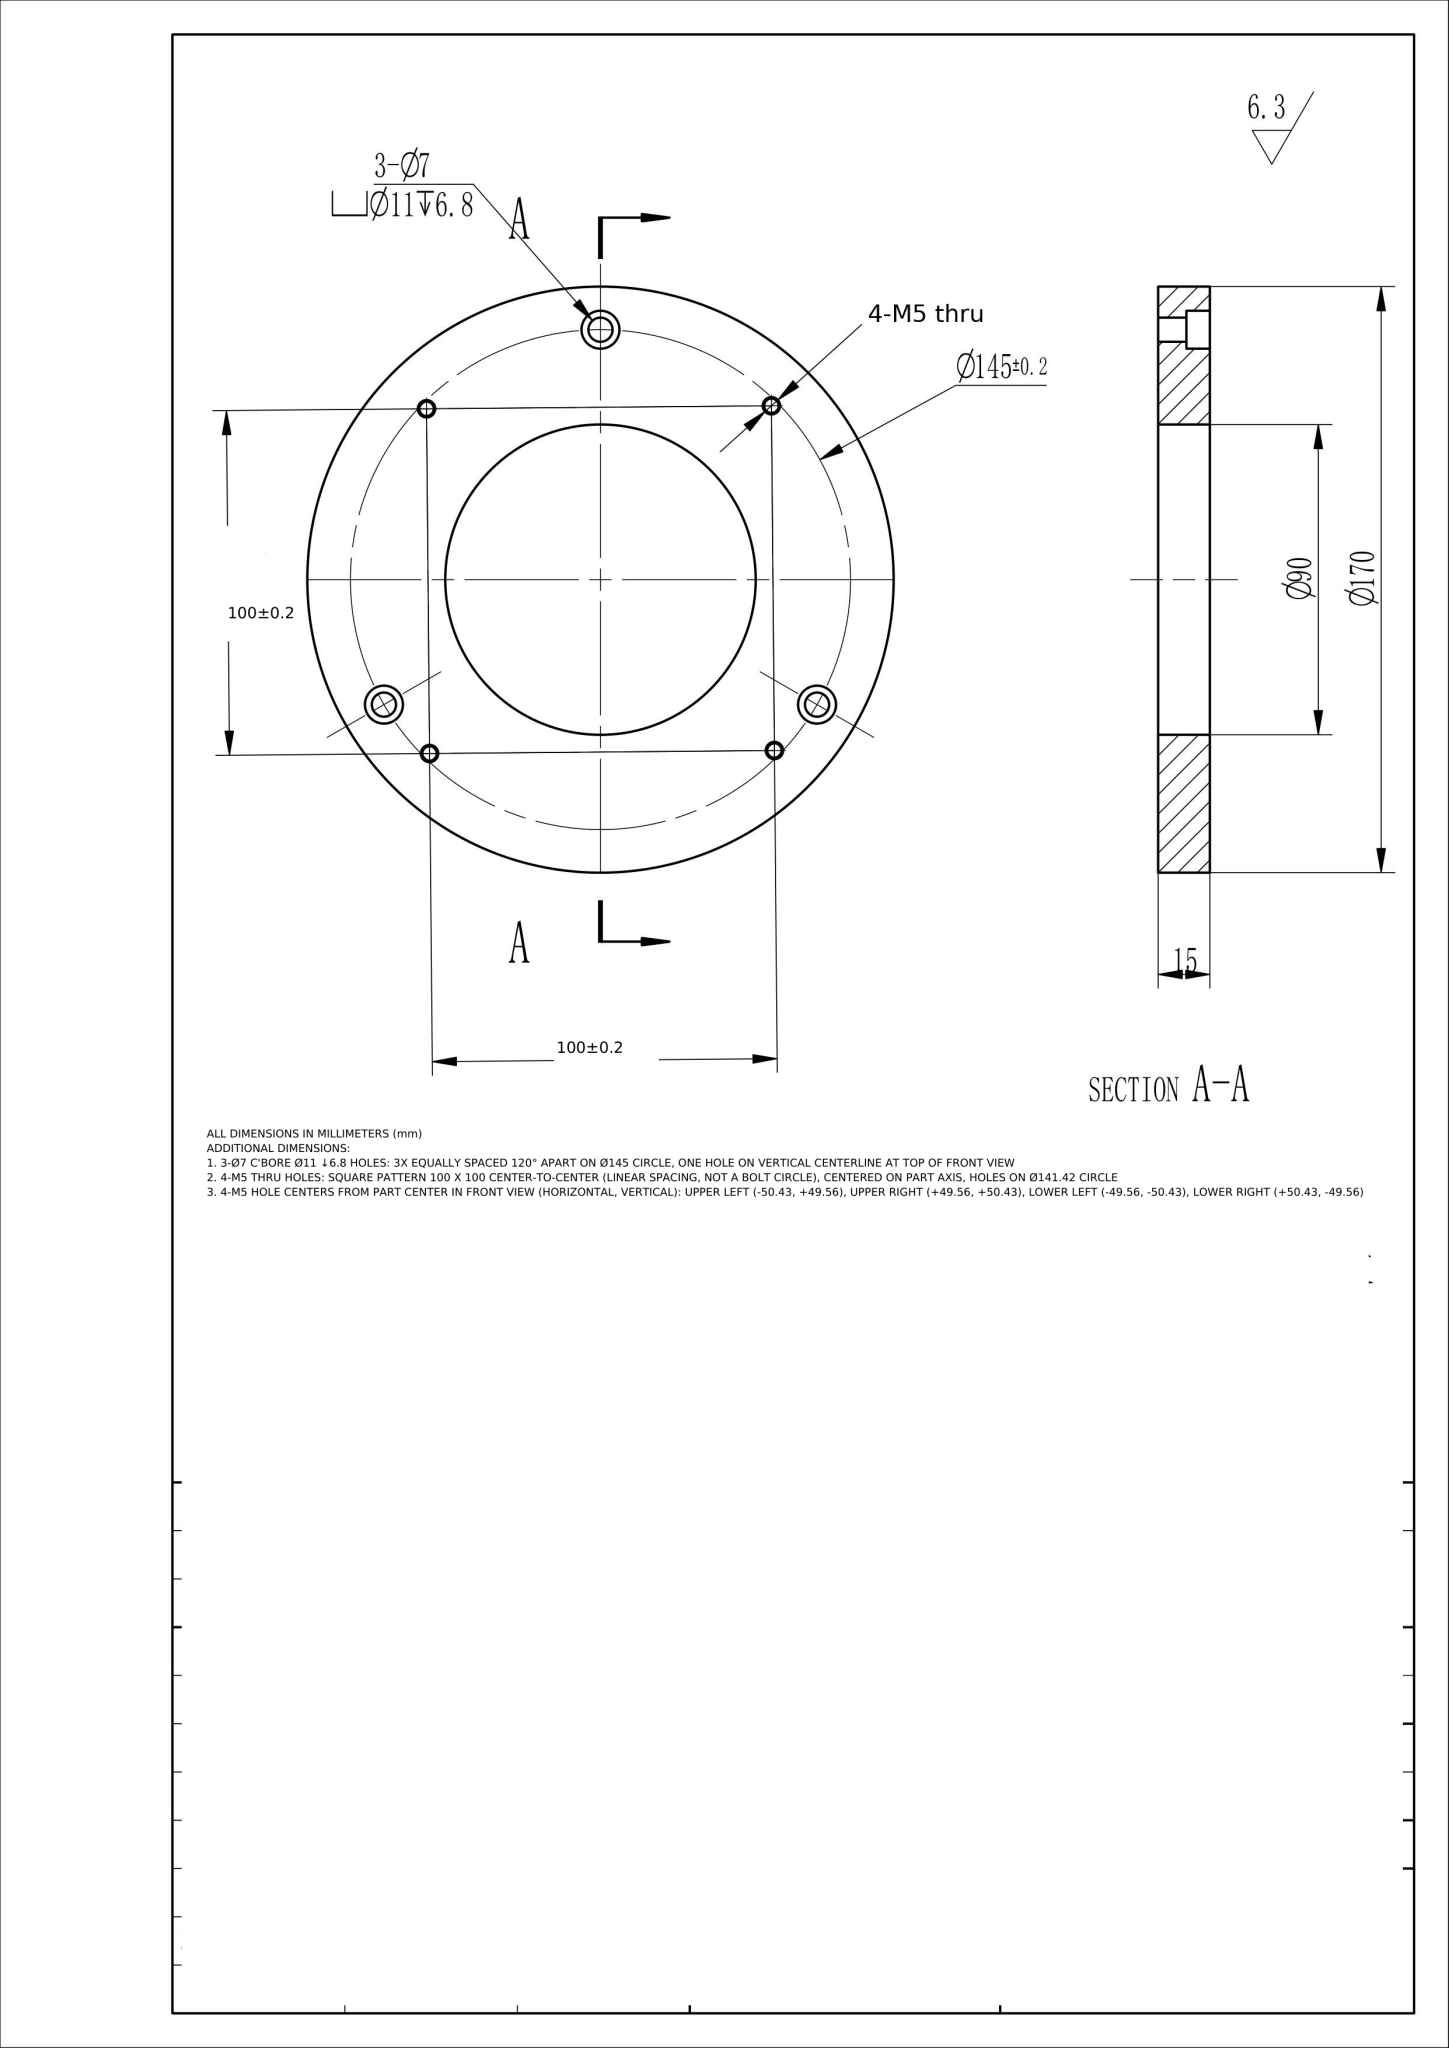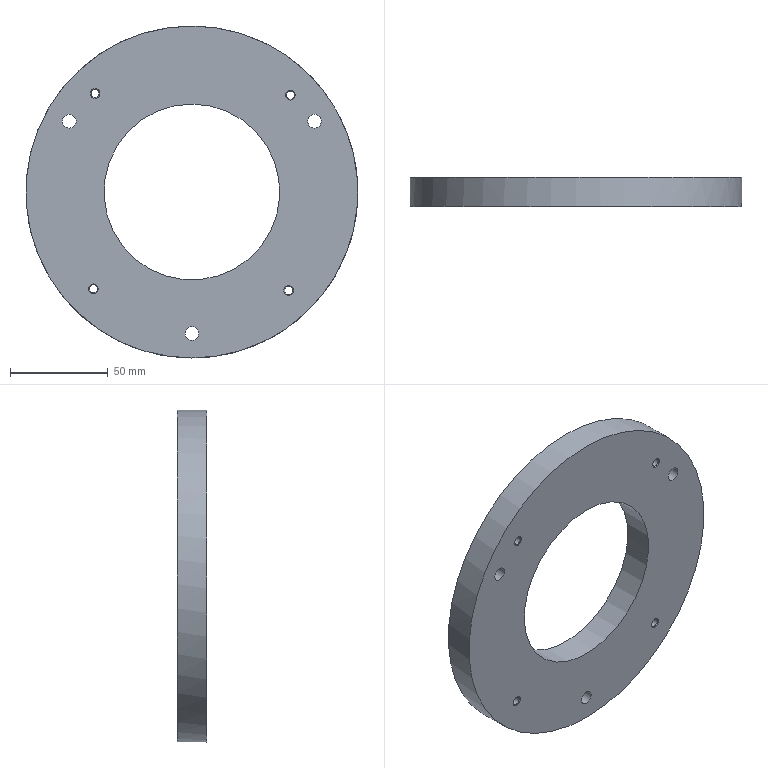Part | NX | mm | 1 solid | 25 faces | box 170 x 15 x 170 mm | volume 241319 mm3 | cylinder 12 | cone 8 | plane 5 | commonest cylinder face diameters 4.2 x4 7 x3 11 x3 170 x1 90 x1
STEP:
#1=CARTESIAN_POINT('',(0.,0.,0.));
#2=DIRECTION('',(0.,0.,1.));
#3=DIRECTION('',(1.,0.,0.));
#4=AXIS2_PLACEMENT_3D('',#1,#2,#3);
#5=(LENGTH_UNIT()NAMED_UNIT(*)SI_UNIT(.MILLI.,.METRE.));
#6=UNCERTAINTY_MEASURE_WITH_UNIT(LENGTH_MEASURE(0.00002),#5,'','');
#7=(NAMED_UNIT(*)PLANE_ANGLE_UNIT()SI_UNIT($,.RADIAN.));
#8=PLANE_ANGLE_MEASURE_WITH_UNIT(PLANE_ANGLE_MEASURE(0.01745),#7);
#9=DIMENSIONAL_EXPONENTS(0.,0.,0.,0.,0.,0.,0.);
#10=(CONVERSION_BASED_UNIT('',#8)NAMED_UNIT(#9)PLANE_ANGLE_UNIT());
#11=(NAMED_UNIT(*)SI_UNIT($,.STERADIAN.)SOLID_ANGLE_UNIT());
#12=(GEOMETRIC_REPRESENTATION_CONTEXT(3)GLOBAL_UNCERTAINTY_ASSIGNED_CONTEXT((#6))GLOBAL_UNIT_ASSIGNED_CONTEXT((#5,#10,#11))REPRESENTATION_CONTEXT('',''));
#13=SHAPE_REPRESENTATION('',(#4),#12);
#14=CARTESIAN_POINT('',(0.,409.,85.));
#15=VERTEX_POINT('',#14);
#16=CARTESIAN_POINT('',(0.,409.,0.));
#17=DIRECTION('',(0.,1.,0.));
#18=DIRECTION('',(0.,0.,1.));
#19=AXIS2_PLACEMENT_3D('',#16,#17,#18);
#20=CIRCLE('',#19,85.);
#21=EDGE_CURVE('',#15,#15,#20,.T.);
#22=ORIENTED_EDGE('',*,*,#21,.T.);
#23=EDGE_LOOP('',(#22));
#24=FACE_BOUND('',#23,.T.);
#25=CARTESIAN_POINT('',(85.,424.,0.));
#26=VERTEX_POINT('',#25);
#27=CARTESIAN_POINT('',(0.,424.,0.));
#28=DIRECTION('',(0.,1.,0.));
#29=DIRECTION('',(1.,0.,0.));
#30=AXIS2_PLACEMENT_3D('',#27,#28,#29);
#31=CIRCLE('',#30,85.);
#32=EDGE_CURVE('',#26,#26,#31,.T.);
#33=ORIENTED_EDGE('',*,*,#32,.F.);
#34=EDGE_LOOP('',(#33));
#35=FACE_BOUND('',#34,.T.);
#36=CARTESIAN_POINT('',(0.,414.,0.));
#37=DIRECTION('',(0.,1.,0.));
#38=DIRECTION('',(0.,0.,1.));
#39=AXIS2_PLACEMENT_3D('',#36,#37,#38);
#40=CYLINDRICAL_SURFACE('',#39,85.);
#41=ADVANCED_FACE('',(#24,#35),#40,.T.);
#42=CARTESIAN_POINT('',(50.434,409.,52.062));
#43=VERTEX_POINT('',#42);
#44=CARTESIAN_POINT('',(50.434,409.,49.562));
#45=DIRECTION('',(0.,1.,0.));
#46=DIRECTION('',(0.,0.,1.));
#47=AXIS2_PLACEMENT_3D('',#44,#45,#46);
#48=CIRCLE('',#47,2.5);
#49=EDGE_CURVE('',#43,#43,#48,.T.);
#50=ORIENTED_EDGE('',*,*,#49,.T.);
#51=EDGE_LOOP('',(#50));
#52=FACE_BOUND('',#51,.T.);
#53=CARTESIAN_POINT('',(49.562,409.,-47.934));
#54=VERTEX_POINT('',#53);
#55=CARTESIAN_POINT('',(49.562,409.,-50.434));
#56=DIRECTION('',(0.,1.,0.));
#57=DIRECTION('',(0.,0.,1.));
#58=AXIS2_PLACEMENT_3D('',#55,#56,#57);
#59=CIRCLE('',#58,2.5);
#60=EDGE_CURVE('',#54,#54,#59,.T.);
#61=ORIENTED_EDGE('',*,*,#60,.T.);
#62=EDGE_LOOP('',(#61));
#63=FACE_BOUND('',#62,.T.);
#64=CARTESIAN_POINT('',(-49.562,409.,52.934));
#65=VERTEX_POINT('',#64);
#66=CARTESIAN_POINT('',(-49.562,409.,50.434));
#67=DIRECTION('',(0.,1.,0.));
#68=DIRECTION('',(0.,0.,1.));
#69=AXIS2_PLACEMENT_3D('',#66,#67,#68);
#70=CIRCLE('',#69,2.5);
#71=EDGE_CURVE('',#65,#65,#70,.T.);
#72=ORIENTED_EDGE('',*,*,#71,.T.);
#73=EDGE_LOOP('',(#72));
#74=FACE_BOUND('',#73,.T.);
#75=CARTESIAN_POINT('',(-50.434,409.,-47.062));
#76=VERTEX_POINT('',#75);
#77=CARTESIAN_POINT('',(-50.434,409.,-49.562));
#78=DIRECTION('',(0.,1.,0.));
#79=DIRECTION('',(0.,0.,1.));
#80=AXIS2_PLACEMENT_3D('',#77,#78,#79);
#81=CIRCLE('',#80,2.5);
#82=EDGE_CURVE('',#76,#76,#81,.T.);
#83=ORIENTED_EDGE('',*,*,#82,.T.);
#84=EDGE_LOOP('',(#83));
#85=FACE_BOUND('',#84,.T.);
#86=CARTESIAN_POINT('',(-0.,409.,45.));
#87=VERTEX_POINT('',#86);
#88=CARTESIAN_POINT('',(-0.,409.,-0.));
#89=DIRECTION('',(0.,-1.,0.));
#90=DIRECTION('',(0.,0.,1.));
#91=AXIS2_PLACEMENT_3D('',#88,#89,#90);
#92=CIRCLE('',#91,45.);
#93=EDGE_CURVE('',#87,#87,#92,.T.);
#94=ORIENTED_EDGE('',*,*,#93,.F.);
#95=EDGE_LOOP('',(#94));
#96=FACE_BOUND('',#95,.T.);
#97=CARTESIAN_POINT('',(62.787,409.,39.75));
#98=VERTEX_POINT('',#97);
#99=CARTESIAN_POINT('',(62.787,409.,36.25));
#100=DIRECTION('',(0.,1.,0.));
#101=DIRECTION('',(0.,0.,1.));
#102=AXIS2_PLACEMENT_3D('',#99,#100,#101);
#103=CIRCLE('',#102,3.5);
#104=EDGE_CURVE('',#98,#98,#103,.T.);
#105=ORIENTED_EDGE('',*,*,#104,.T.);
#106=EDGE_LOOP('',(#105));
#107=FACE_BOUND('',#106,.T.);
#108=CARTESIAN_POINT('',(-62.787,409.,39.75));
#109=VERTEX_POINT('',#108);
#110=CARTESIAN_POINT('',(-62.787,409.,36.25));
#111=DIRECTION('',(0.,1.,0.));
#112=DIRECTION('',(0.,0.,1.));
#113=AXIS2_PLACEMENT_3D('',#110,#111,#112);
#114=CIRCLE('',#113,3.5);
#115=EDGE_CURVE('',#109,#109,#114,.T.);
#116=ORIENTED_EDGE('',*,*,#115,.T.);
#117=EDGE_LOOP('',(#116));
#118=FACE_BOUND('',#117,.T.);
#119=CARTESIAN_POINT('',(0.,409.,-69.));
#120=VERTEX_POINT('',#119);
#121=CARTESIAN_POINT('',(0.,409.,-72.5));
#122=DIRECTION('',(0.,1.,0.));
#123=DIRECTION('',(0.,0.,1.));
#124=AXIS2_PLACEMENT_3D('',#121,#122,#123);
#125=CIRCLE('',#124,3.5);
#126=EDGE_CURVE('',#120,#120,#125,.T.);
#127=ORIENTED_EDGE('',*,*,#126,.T.);
#128=EDGE_LOOP('',(#127));
#129=FACE_BOUND('',#128,.T.);
#130=ORIENTED_EDGE('',*,*,#21,.F.);
#131=EDGE_LOOP('',(#130));
#132=FACE_BOUND('',#131,.T.);
#133=CARTESIAN_POINT('',(0.,409.,0.));
#134=DIRECTION('',(0.,1.,0.));
#135=DIRECTION('',(0.,0.,1.));
#136=AXIS2_PLACEMENT_3D('',#133,#134,#135);
#137=PLANE('',#136);
#138=ADVANCED_FACE('',(#52,#63,#74,#85,#96,#107,#118,#129,#132),#137,.F.);
#139=CARTESIAN_POINT('',(50.434,424.,52.062));
#140=VERTEX_POINT('',#139);
#141=CARTESIAN_POINT('',(50.434,424.,49.562));
#142=DIRECTION('',(0.,-1.,0.));
#143=DIRECTION('',(0.,0.,1.));
#144=AXIS2_PLACEMENT_3D('',#141,#142,#143);
#145=CIRCLE('',#144,2.5);
#146=EDGE_CURVE('',#140,#140,#145,.T.);
#147=ORIENTED_EDGE('',*,*,#146,.T.);
#148=EDGE_LOOP('',(#147));
#149=FACE_BOUND('',#148,.T.);
#150=CARTESIAN_POINT('',(49.562,424.,-47.934));
#151=VERTEX_POINT('',#150);
#152=CARTESIAN_POINT('',(49.562,424.,-50.434));
#153=DIRECTION('',(0.,-1.,0.));
#154=DIRECTION('',(0.,0.,1.));
#155=AXIS2_PLACEMENT_3D('',#152,#153,#154);
#156=CIRCLE('',#155,2.5);
#157=EDGE_CURVE('',#151,#151,#156,.T.);
#158=ORIENTED_EDGE('',*,*,#157,.T.);
#159=EDGE_LOOP('',(#158));
#160=FACE_BOUND('',#159,.T.);
#161=CARTESIAN_POINT('',(-49.562,424.,52.934));
#162=VERTEX_POINT('',#161);
#163=CARTESIAN_POINT('',(-49.562,424.,50.434));
#164=DIRECTION('',(0.,-1.,0.));
#165=DIRECTION('',(0.,0.,1.));
#166=AXIS2_PLACEMENT_3D('',#163,#164,#165);
#167=CIRCLE('',#166,2.5);
#168=EDGE_CURVE('',#162,#162,#167,.T.);
#169=ORIENTED_EDGE('',*,*,#168,.T.);
#170=EDGE_LOOP('',(#169));
#171=FACE_BOUND('',#170,.T.);
#172=CARTESIAN_POINT('',(-50.434,424.,-47.062));
#173=VERTEX_POINT('',#172);
#174=CARTESIAN_POINT('',(-50.434,424.,-49.562));
#175=DIRECTION('',(0.,-1.,0.));
#176=DIRECTION('',(0.,0.,1.));
#177=AXIS2_PLACEMENT_3D('',#174,#175,#176);
#178=CIRCLE('',#177,2.5);
#179=EDGE_CURVE('',#173,#173,#178,.T.);
#180=ORIENTED_EDGE('',*,*,#179,.T.);
#181=EDGE_LOOP('',(#180));
#182=FACE_BOUND('',#181,.T.);
#183=CARTESIAN_POINT('',(-0.,424.,45.));
#184=VERTEX_POINT('',#183);
#185=CARTESIAN_POINT('',(-0.,424.,-0.));
#186=DIRECTION('',(0.,-1.,0.));
#187=DIRECTION('',(0.,0.,1.));
#188=AXIS2_PLACEMENT_3D('',#185,#186,#187);
#189=CIRCLE('',#188,45.);
#190=EDGE_CURVE('',#184,#184,#189,.T.);
#191=ORIENTED_EDGE('',*,*,#190,.T.);
#192=EDGE_LOOP('',(#191));
#193=FACE_BOUND('',#192,.T.);
#194=CARTESIAN_POINT('',(62.787,424.,30.75));
#195=VERTEX_POINT('',#194);
#196=CARTESIAN_POINT('',(62.787,424.,36.25));
#197=DIRECTION('',(0.,-1.,0.));
#198=DIRECTION('',(0.,0.,-1.));
#199=AXIS2_PLACEMENT_3D('',#196,#197,#198);
#200=CIRCLE('',#199,5.5);
#201=EDGE_CURVE('',#195,#195,#200,.T.);
#202=ORIENTED_EDGE('',*,*,#201,.T.);
#203=EDGE_LOOP('',(#202));
#204=FACE_BOUND('',#203,.T.);
#205=CARTESIAN_POINT('',(-62.787,424.,30.75));
#206=VERTEX_POINT('',#205);
#207=CARTESIAN_POINT('',(-62.787,424.,36.25));
#208=DIRECTION('',(0.,-1.,0.));
#209=DIRECTION('',(0.,0.,-1.));
#210=AXIS2_PLACEMENT_3D('',#207,#208,#209);
#211=CIRCLE('',#210,5.5);
#212=EDGE_CURVE('',#206,#206,#211,.T.);
#213=ORIENTED_EDGE('',*,*,#212,.T.);
#214=EDGE_LOOP('',(#213));
#215=FACE_BOUND('',#214,.T.);
#216=CARTESIAN_POINT('',(0.,424.,-78.));
#217=VERTEX_POINT('',#216);
#218=CARTESIAN_POINT('',(0.,424.,-72.5));
#219=DIRECTION('',(0.,-1.,0.));
#220=DIRECTION('',(0.,0.,-1.));
#221=AXIS2_PLACEMENT_3D('',#218,#219,#220);
#222=CIRCLE('',#221,5.5);
#223=EDGE_CURVE('',#217,#217,#222,.T.);
#224=ORIENTED_EDGE('',*,*,#223,.T.);
#225=EDGE_LOOP('',(#224));
#226=FACE_BOUND('',#225,.T.);
#227=ORIENTED_EDGE('',*,*,#32,.T.);
#228=EDGE_LOOP('',(#227));
#229=FACE_BOUND('',#228,.T.);
#230=CARTESIAN_POINT('',(0.,424.,0.));
#231=DIRECTION('',(0.,1.,0.));
#232=DIRECTION('',(0.,0.,1.));
#233=AXIS2_PLACEMENT_3D('',#230,#231,#232);
#234=PLANE('',#233);
#235=ADVANCED_FACE('',(#149,#160,#171,#182,#193,#204,#215,#226,#229),#234,.T.);
#236=CARTESIAN_POINT('',(0.,417.2,-76.));
#237=VERTEX_POINT('',#236);
#238=CARTESIAN_POINT('',(0.,417.2,-72.5));
#239=DIRECTION('',(0.,1.,0.));
#240=DIRECTION('',(0.,0.,-1.));
#241=AXIS2_PLACEMENT_3D('',#238,#239,#240);
#242=CIRCLE('',#241,3.5);
#243=EDGE_CURVE('',#237,#237,#242,.T.);
#244=ORIENTED_EDGE('',*,*,#243,.T.);
#245=EDGE_LOOP('',(#244));
#246=FACE_BOUND('',#245,.T.);
#247=ORIENTED_EDGE('',*,*,#126,.F.);
#248=EDGE_LOOP('',(#247));
#249=FACE_BOUND('',#248,.T.);
#250=CARTESIAN_POINT('',(0.,409.,-72.5));
#251=DIRECTION('',(0.,-1.,0.));
#252=DIRECTION('',(0.,0.,-1.));
#253=AXIS2_PLACEMENT_3D('',#250,#251,#252);
#254=CYLINDRICAL_SURFACE('',#253,3.5);
#255=ADVANCED_FACE('',(#246,#249),#254,.F.);
#256=ORIENTED_EDGE('',*,*,#243,.F.);
#257=EDGE_LOOP('',(#256));
#258=FACE_BOUND('',#257,.T.);
#259=CARTESIAN_POINT('',(0.,417.2,-78.));
#260=VERTEX_POINT('',#259);
#261=CARTESIAN_POINT('',(0.,417.2,-72.5));
#262=DIRECTION('',(0.,1.,0.));
#263=DIRECTION('',(0.,0.,-1.));
#264=AXIS2_PLACEMENT_3D('',#261,#262,#263);
#265=CIRCLE('',#264,5.5);
#266=EDGE_CURVE('',#260,#260,#265,.T.);
#267=ORIENTED_EDGE('',*,*,#266,.T.);
#268=EDGE_LOOP('',(#267));
#269=FACE_BOUND('',#268,.T.);
#270=CARTESIAN_POINT('',(0.,417.2,-72.5));
#271=DIRECTION('',(0.,-1.,0.));
#272=DIRECTION('',(0.,0.,-1.));
#273=AXIS2_PLACEMENT_3D('',#270,#271,#272);
#274=PLANE('',#273);
#275=ADVANCED_FACE('',(#258,#269),#274,.F.);
#276=ORIENTED_EDGE('',*,*,#266,.F.);
#277=EDGE_LOOP('',(#276));
#278=FACE_BOUND('',#277,.T.);
#279=ORIENTED_EDGE('',*,*,#223,.F.);
#280=EDGE_LOOP('',(#279));
#281=FACE_BOUND('',#280,.T.);
#282=CARTESIAN_POINT('',(0.,424.,-72.5));
#283=DIRECTION('',(0.,-1.,0.));
#284=DIRECTION('',(0.,0.,-1.));
#285=AXIS2_PLACEMENT_3D('',#282,#283,#284);
#286=CYLINDRICAL_SURFACE('',#285,5.5);
#287=ADVANCED_FACE('',(#278,#281),#286,.F.);
#288=CARTESIAN_POINT('',(-62.787,417.2,32.75));
#289=VERTEX_POINT('',#288);
#290=CARTESIAN_POINT('',(-62.787,417.2,36.25));
#291=DIRECTION('',(0.,1.,0.));
#292=DIRECTION('',(0.,0.,-1.));
#293=AXIS2_PLACEMENT_3D('',#290,#291,#292);
#294=CIRCLE('',#293,3.5);
#295=EDGE_CURVE('',#289,#289,#294,.T.);
#296=ORIENTED_EDGE('',*,*,#295,.T.);
#297=EDGE_LOOP('',(#296));
#298=FACE_BOUND('',#297,.T.);
#299=ORIENTED_EDGE('',*,*,#115,.F.);
#300=EDGE_LOOP('',(#299));
#301=FACE_BOUND('',#300,.T.);
#302=CARTESIAN_POINT('',(-62.787,409.,36.25));
#303=DIRECTION('',(0.,-1.,0.));
#304=DIRECTION('',(0.,0.,-1.));
#305=AXIS2_PLACEMENT_3D('',#302,#303,#304);
#306=CYLINDRICAL_SURFACE('',#305,3.5);
#307=ADVANCED_FACE('',(#298,#301),#306,.F.);
#308=ORIENTED_EDGE('',*,*,#295,.F.);
#309=EDGE_LOOP('',(#308));
#310=FACE_BOUND('',#309,.T.);
#311=CARTESIAN_POINT('',(-62.787,417.2,30.75));
#312=VERTEX_POINT('',#311);
#313=CARTESIAN_POINT('',(-62.787,417.2,36.25));
#314=DIRECTION('',(0.,1.,0.));
#315=DIRECTION('',(0.,0.,-1.));
#316=AXIS2_PLACEMENT_3D('',#313,#314,#315);
#317=CIRCLE('',#316,5.5);
#318=EDGE_CURVE('',#312,#312,#317,.T.);
#319=ORIENTED_EDGE('',*,*,#318,.T.);
#320=EDGE_LOOP('',(#319));
#321=FACE_BOUND('',#320,.T.);
#322=CARTESIAN_POINT('',(-62.787,417.2,36.25));
#323=DIRECTION('',(0.,-1.,0.));
#324=DIRECTION('',(0.,0.,-1.));
#325=AXIS2_PLACEMENT_3D('',#322,#323,#324);
#326=PLANE('',#325);
#327=ADVANCED_FACE('',(#310,#321),#326,.F.);
#328=ORIENTED_EDGE('',*,*,#318,.F.);
#329=EDGE_LOOP('',(#328));
#330=FACE_BOUND('',#329,.T.);
#331=ORIENTED_EDGE('',*,*,#212,.F.);
#332=EDGE_LOOP('',(#331));
#333=FACE_BOUND('',#332,.T.);
#334=CARTESIAN_POINT('',(-62.787,424.,36.25));
#335=DIRECTION('',(0.,-1.,0.));
#336=DIRECTION('',(0.,0.,-1.));
#337=AXIS2_PLACEMENT_3D('',#334,#335,#336);
#338=CYLINDRICAL_SURFACE('',#337,5.5);
#339=ADVANCED_FACE('',(#330,#333),#338,.F.);
#340=CARTESIAN_POINT('',(62.787,417.2,32.75));
#341=VERTEX_POINT('',#340);
#342=CARTESIAN_POINT('',(62.787,417.2,36.25));
#343=DIRECTION('',(0.,1.,0.));
#344=DIRECTION('',(0.,0.,-1.));
#345=AXIS2_PLACEMENT_3D('',#342,#343,#344);
#346=CIRCLE('',#345,3.5);
#347=EDGE_CURVE('',#341,#341,#346,.T.);
#348=ORIENTED_EDGE('',*,*,#347,.T.);
#349=EDGE_LOOP('',(#348));
#350=FACE_BOUND('',#349,.T.);
#351=ORIENTED_EDGE('',*,*,#104,.F.);
#352=EDGE_LOOP('',(#351));
#353=FACE_BOUND('',#352,.T.);
#354=CARTESIAN_POINT('',(62.787,409.,36.25));
#355=DIRECTION('',(0.,-1.,0.));
#356=DIRECTION('',(0.,0.,-1.));
#357=AXIS2_PLACEMENT_3D('',#354,#355,#356);
#358=CYLINDRICAL_SURFACE('',#357,3.5);
#359=ADVANCED_FACE('',(#350,#353),#358,.F.);
#360=ORIENTED_EDGE('',*,*,#347,.F.);
#361=EDGE_LOOP('',(#360));
#362=FACE_BOUND('',#361,.T.);
#363=CARTESIAN_POINT('',(62.787,417.2,30.75));
#364=VERTEX_POINT('',#363);
#365=CARTESIAN_POINT('',(62.787,417.2,36.25));
#366=DIRECTION('',(0.,1.,0.));
#367=DIRECTION('',(0.,0.,-1.));
#368=AXIS2_PLACEMENT_3D('',#365,#366,#367);
#369=CIRCLE('',#368,5.5);
#370=EDGE_CURVE('',#364,#364,#369,.T.);
#371=ORIENTED_EDGE('',*,*,#370,.T.);
#372=EDGE_LOOP('',(#371));
#373=FACE_BOUND('',#372,.T.);
#374=CARTESIAN_POINT('',(62.787,417.2,36.25));
#375=DIRECTION('',(0.,-1.,0.));
#376=DIRECTION('',(0.,0.,-1.));
#377=AXIS2_PLACEMENT_3D('',#374,#375,#376);
#378=PLANE('',#377);
#379=ADVANCED_FACE('',(#362,#373),#378,.F.);
#380=ORIENTED_EDGE('',*,*,#370,.F.);
#381=EDGE_LOOP('',(#380));
#382=FACE_BOUND('',#381,.T.);
#383=ORIENTED_EDGE('',*,*,#201,.F.);
#384=EDGE_LOOP('',(#383));
#385=FACE_BOUND('',#384,.T.);
#386=CARTESIAN_POINT('',(62.787,424.,36.25));
#387=DIRECTION('',(0.,-1.,0.));
#388=DIRECTION('',(0.,0.,-1.));
#389=AXIS2_PLACEMENT_3D('',#386,#387,#388);
#390=CYLINDRICAL_SURFACE('',#389,5.5);
#391=ADVANCED_FACE('',(#382,#385),#390,.F.);
#392=ORIENTED_EDGE('',*,*,#190,.F.);
#393=EDGE_LOOP('',(#392));
#394=FACE_BOUND('',#393,.T.);
#395=ORIENTED_EDGE('',*,*,#93,.T.);
#396=EDGE_LOOP('',(#395));
#397=FACE_BOUND('',#396,.T.);
#398=CARTESIAN_POINT('',(-0.,434.,-0.));
#399=DIRECTION('',(0.,-1.,0.));
#400=DIRECTION('',(0.,0.,-1.));
#401=AXIS2_PLACEMENT_3D('',#398,#399,#400);
#402=CYLINDRICAL_SURFACE('',#401,45.);
#403=ADVANCED_FACE('',(#394,#397),#402,.F.);
#404=CARTESIAN_POINT('',(-50.434,409.4,-47.462));
#405=VERTEX_POINT('',#404);
#406=CARTESIAN_POINT('',(-50.434,409.4,-49.562));
#407=DIRECTION('',(0.,-1.,0.));
#408=DIRECTION('',(0.,0.,1.));
#409=AXIS2_PLACEMENT_3D('',#406,#407,#408);
#410=CIRCLE('',#409,2.1);
#411=EDGE_CURVE('',#405,#405,#410,.T.);
#412=ORIENTED_EDGE('',*,*,#411,.T.);
#413=EDGE_LOOP('',(#412));
#414=FACE_BOUND('',#413,.T.);
#415=CARTESIAN_POINT('',(-50.434,423.6,-47.462));
#416=VERTEX_POINT('',#415);
#417=CARTESIAN_POINT('',(-50.434,423.6,-49.562));
#418=DIRECTION('',(0.,1.,0.));
#419=DIRECTION('',(0.,0.,1.));
#420=AXIS2_PLACEMENT_3D('',#417,#418,#419);
#421=CIRCLE('',#420,2.1);
#422=EDGE_CURVE('',#416,#416,#421,.T.);
#423=ORIENTED_EDGE('',*,*,#422,.T.);
#424=EDGE_LOOP('',(#423));
#425=FACE_BOUND('',#424,.T.);
#426=CARTESIAN_POINT('',(-50.434,424.,-49.562));
#427=DIRECTION('',(0.,-1.,0.));
#428=DIRECTION('',(0.,0.,-1.));
#429=AXIS2_PLACEMENT_3D('',#426,#427,#428);
#430=CYLINDRICAL_SURFACE('',#429,2.1);
#431=ADVANCED_FACE('',(#414,#425),#430,.F.);
#432=ORIENTED_EDGE('',*,*,#422,.F.);
#433=EDGE_LOOP('',(#432));
#434=FACE_BOUND('',#433,.T.);
#435=ORIENTED_EDGE('',*,*,#179,.F.);
#436=EDGE_LOOP('',(#435));
#437=FACE_BOUND('',#436,.T.);
#438=CARTESIAN_POINT('',(-50.434,424.,-49.562));
#439=DIRECTION('',(0.,1.,0.));
#440=DIRECTION('',(0.,0.,1.));
#441=AXIS2_PLACEMENT_3D('',#438,#439,#440);
#442=CONICAL_SURFACE('',#441,2.5,45.);
#443=ADVANCED_FACE('',(#434,#437),#442,.F.);
#444=ORIENTED_EDGE('',*,*,#411,.F.);
#445=EDGE_LOOP('',(#444));
#446=FACE_BOUND('',#445,.T.);
#447=ORIENTED_EDGE('',*,*,#82,.F.);
#448=EDGE_LOOP('',(#447));
#449=FACE_BOUND('',#448,.T.);
#450=CARTESIAN_POINT('',(-50.434,409.,-49.562));
#451=DIRECTION('',(0.,-1.,0.));
#452=DIRECTION('',(0.,-0.,-1.));
#453=AXIS2_PLACEMENT_3D('',#450,#451,#452);
#454=CONICAL_SURFACE('',#453,2.5,45.);
#455=ADVANCED_FACE('',(#446,#449),#454,.F.);
#456=CARTESIAN_POINT('',(-49.562,409.4,52.534));
#457=VERTEX_POINT('',#456);
#458=CARTESIAN_POINT('',(-49.562,409.4,50.434));
#459=DIRECTION('',(0.,-1.,0.));
#460=DIRECTION('',(0.,0.,1.));
#461=AXIS2_PLACEMENT_3D('',#458,#459,#460);
#462=CIRCLE('',#461,2.1);
#463=EDGE_CURVE('',#457,#457,#462,.T.);
#464=ORIENTED_EDGE('',*,*,#463,.T.);
#465=EDGE_LOOP('',(#464));
#466=FACE_BOUND('',#465,.T.);
#467=CARTESIAN_POINT('',(-49.562,423.6,52.534));
#468=VERTEX_POINT('',#467);
#469=CARTESIAN_POINT('',(-49.562,423.6,50.434));
#470=DIRECTION('',(0.,1.,0.));
#471=DIRECTION('',(0.,0.,1.));
#472=AXIS2_PLACEMENT_3D('',#469,#470,#471);
#473=CIRCLE('',#472,2.1);
#474=EDGE_CURVE('',#468,#468,#473,.T.);
#475=ORIENTED_EDGE('',*,*,#474,.T.);
#476=EDGE_LOOP('',(#475));
#477=FACE_BOUND('',#476,.T.);
#478=CARTESIAN_POINT('',(-49.562,424.,50.434));
#479=DIRECTION('',(0.,-1.,0.));
#480=DIRECTION('',(0.,0.,-1.));
#481=AXIS2_PLACEMENT_3D('',#478,#479,#480);
#482=CYLINDRICAL_SURFACE('',#481,2.1);
#483=ADVANCED_FACE('',(#466,#477),#482,.F.);
#484=ORIENTED_EDGE('',*,*,#474,.F.);
#485=EDGE_LOOP('',(#484));
#486=FACE_BOUND('',#485,.T.);
#487=ORIENTED_EDGE('',*,*,#168,.F.);
#488=EDGE_LOOP('',(#487));
#489=FACE_BOUND('',#488,.T.);
#490=CARTESIAN_POINT('',(-49.562,424.,50.434));
#491=DIRECTION('',(0.,1.,0.));
#492=DIRECTION('',(0.,0.,1.));
#493=AXIS2_PLACEMENT_3D('',#490,#491,#492);
#494=CONICAL_SURFACE('',#493,2.5,45.);
#495=ADVANCED_FACE('',(#486,#489),#494,.F.);
#496=ORIENTED_EDGE('',*,*,#463,.F.);
#497=EDGE_LOOP('',(#496));
#498=FACE_BOUND('',#497,.T.);
#499=ORIENTED_EDGE('',*,*,#71,.F.);
#500=EDGE_LOOP('',(#499));
#501=FACE_BOUND('',#500,.T.);
#502=CARTESIAN_POINT('',(-49.562,409.,50.434));
#503=DIRECTION('',(0.,-1.,0.));
#504=DIRECTION('',(0.,-0.,-1.));
#505=AXIS2_PLACEMENT_3D('',#502,#503,#504);
#506=CONICAL_SURFACE('',#505,2.5,45.);
#507=ADVANCED_FACE('',(#498,#501),#506,.F.);
#508=CARTESIAN_POINT('',(49.562,409.4,-48.334));
#509=VERTEX_POINT('',#508);
#510=CARTESIAN_POINT('',(49.562,409.4,-50.434));
#511=DIRECTION('',(0.,-1.,0.));
#512=DIRECTION('',(0.,0.,1.));
#513=AXIS2_PLACEMENT_3D('',#510,#511,#512);
#514=CIRCLE('',#513,2.1);
#515=EDGE_CURVE('',#509,#509,#514,.T.);
#516=ORIENTED_EDGE('',*,*,#515,.T.);
#517=EDGE_LOOP('',(#516));
#518=FACE_BOUND('',#517,.T.);
#519=CARTESIAN_POINT('',(49.562,423.6,-48.334));
#520=VERTEX_POINT('',#519);
#521=CARTESIAN_POINT('',(49.562,423.6,-50.434));
#522=DIRECTION('',(0.,1.,0.));
#523=DIRECTION('',(0.,0.,1.));
#524=AXIS2_PLACEMENT_3D('',#521,#522,#523);
#525=CIRCLE('',#524,2.1);
#526=EDGE_CURVE('',#520,#520,#525,.T.);
#527=ORIENTED_EDGE('',*,*,#526,.T.);
#528=EDGE_LOOP('',(#527));
#529=FACE_BOUND('',#528,.T.);
#530=CARTESIAN_POINT('',(49.562,424.,-50.434));
#531=DIRECTION('',(0.,-1.,0.));
#532=DIRECTION('',(0.,0.,-1.));
#533=AXIS2_PLACEMENT_3D('',#530,#531,#532);
#534=CYLINDRICAL_SURFACE('',#533,2.1);
#535=ADVANCED_FACE('',(#518,#529),#534,.F.);
#536=ORIENTED_EDGE('',*,*,#526,.F.);
#537=EDGE_LOOP('',(#536));
#538=FACE_BOUND('',#537,.T.);
#539=ORIENTED_EDGE('',*,*,#157,.F.);
#540=EDGE_LOOP('',(#539));
#541=FACE_BOUND('',#540,.T.);
#542=CARTESIAN_POINT('',(49.562,424.,-50.434));
#543=DIRECTION('',(0.,1.,0.));
#544=DIRECTION('',(0.,0.,1.));
#545=AXIS2_PLACEMENT_3D('',#542,#543,#544);
#546=CONICAL_SURFACE('',#545,2.5,45.);
#547=ADVANCED_FACE('',(#538,#541),#546,.F.);
#548=ORIENTED_EDGE('',*,*,#515,.F.);
#549=EDGE_LOOP('',(#548));
#550=FACE_BOUND('',#549,.T.);
#551=ORIENTED_EDGE('',*,*,#60,.F.);
#552=EDGE_LOOP('',(#551));
#553=FACE_BOUND('',#552,.T.);
#554=CARTESIAN_POINT('',(49.562,409.,-50.434));
#555=DIRECTION('',(0.,-1.,0.));
#556=DIRECTION('',(0.,-0.,-1.));
#557=AXIS2_PLACEMENT_3D('',#554,#555,#556);
#558=CONICAL_SURFACE('',#557,2.5,45.);
#559=ADVANCED_FACE('',(#550,#553),#558,.F.);
#560=CARTESIAN_POINT('',(50.434,409.4,51.662));
#561=VERTEX_POINT('',#560);
#562=CARTESIAN_POINT('',(50.434,409.4,49.562));
#563=DIRECTION('',(0.,-1.,0.));
#564=DIRECTION('',(0.,0.,1.));
#565=AXIS2_PLACEMENT_3D('',#562,#563,#564);
#566=CIRCLE('',#565,2.1);
#567=EDGE_CURVE('',#561,#561,#566,.T.);
#568=ORIENTED_EDGE('',*,*,#567,.T.);
#569=EDGE_LOOP('',(#568));
#570=FACE_BOUND('',#569,.T.);
#571=CARTESIAN_POINT('',(50.434,423.6,51.662));
#572=VERTEX_POINT('',#571);
#573=CARTESIAN_POINT('',(50.434,423.6,49.562));
#574=DIRECTION('',(0.,1.,0.));
#575=DIRECTION('',(0.,0.,1.));
#576=AXIS2_PLACEMENT_3D('',#573,#574,#575);
#577=CIRCLE('',#576,2.1);
#578=EDGE_CURVE('',#572,#572,#577,.T.);
#579=ORIENTED_EDGE('',*,*,#578,.T.);
#580=EDGE_LOOP('',(#579));
#581=FACE_BOUND('',#580,.T.);
#582=CARTESIAN_POINT('',(50.434,424.,49.562));
#583=DIRECTION('',(0.,-1.,0.));
#584=DIRECTION('',(0.,0.,-1.));
#585=AXIS2_PLACEMENT_3D('',#582,#583,#584);
#586=CYLINDRICAL_SURFACE('',#585,2.1);
#587=ADVANCED_FACE('',(#570,#581),#586,.F.);
#588=ORIENTED_EDGE('',*,*,#578,.F.);
#589=EDGE_LOOP('',(#588));
#590=FACE_BOUND('',#589,.T.);
#591=ORIENTED_EDGE('',*,*,#146,.F.);
#592=EDGE_LOOP('',(#591));
#593=FACE_BOUND('',#592,.T.);
#594=CARTESIAN_POINT('',(50.434,424.,49.562));
#595=DIRECTION('',(0.,1.,0.));
#596=DIRECTION('',(0.,0.,1.));
#597=AXIS2_PLACEMENT_3D('',#594,#595,#596);
#598=CONICAL_SURFACE('',#597,2.5,45.);
#599=ADVANCED_FACE('',(#590,#593),#598,.F.);
#600=ORIENTED_EDGE('',*,*,#567,.F.);
#601=EDGE_LOOP('',(#600));
#602=FACE_BOUND('',#601,.T.);
#603=ORIENTED_EDGE('',*,*,#49,.F.);
#604=EDGE_LOOP('',(#603));
#605=FACE_BOUND('',#604,.T.);
#606=CARTESIAN_POINT('',(50.434,409.,49.562));
#607=DIRECTION('',(0.,-1.,0.));
#608=DIRECTION('',(0.,-0.,-1.));
#609=AXIS2_PLACEMENT_3D('',#606,#607,#608);
#610=CONICAL_SURFACE('',#609,2.5,45.);
#611=ADVANCED_FACE('',(#602,#605),#610,.F.);
#612=CLOSED_SHELL('',(#41,#138,#235,#255,#275,#287,#307,#327,#339,#359,#379,#391,#403,#431,#443,#455,#483,#495,#507,#535,#547,#559,#587,#599,#611));
#613=MANIFOLD_SOLID_BREP('',#612);
#614=ADVANCED_BREP_SHAPE_REPRESENTATION('',(#613),#12);
#615=SHAPE_REPRESENTATION_RELATIONSHIP('','',#13,#614);
#616=PRESENTATION_LAYER_ASSIGNMENT('','',(#613));
#617=COLOUR_RGB('',1.,0.6,0.);
#618=FILL_AREA_STYLE_COLOUR('',#617);
#619=FILL_AREA_STYLE('',(#618));
#620=SURFACE_STYLE_FILL_AREA(#619);
#621=SURFACE_SIDE_STYLE('',(#620));
#622=SURFACE_STYLE_USAGE(.BOTH.,#621);
#623=PRESENTATION_STYLE_ASSIGNMENT((#622));
#624=STYLED_ITEM('',(#623),#613);
#625=MECHANICAL_DESIGN_GEOMETRIC_PRESENTATION_REPRESENTATION('',(#624),#12);